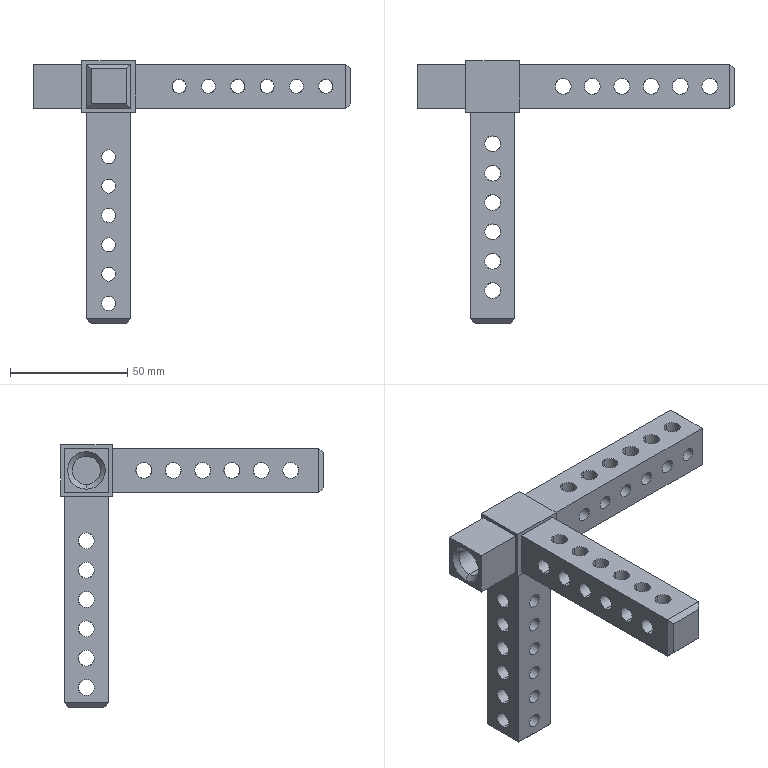Component | SolidWorks | CabinetFrameWeldmentDrawingPG50-01-00-1_FrameConnectionTee1(PG50-01-103-1 | 1 solid | 168 faces | box 135 x 112 x 112 mm | volume 94075 mm3 | cylinder 122 | plane 44 | cone 2 | commonest cylinder face diameters 6.8 x72 6 x48 12 x2 | material AISI 1045 Steel, cold drawn
build123d program:
from build123d import *

# Parameters (mm, degrees)
BOSS_EXTRUDE1_DEPTH      = 9.5
SKETCH2_W                = 19
SKETCH2_H                = 19
BOSS_EXTRUDE2_DEPTH      = 91.5
SKETCH3_W                = 19
SKETCH3_H                = 19
BOSS_EXTRUDE3_DEPTH      = 22.5
SKETCH4_R                = 6
CUT_EXTRUDE1_2_DEPTH     = 20
CHAMFER1_SIZE            = 2
BOSS_EXTRUDE4_DEPTH      = 1.5
BOSS_EXTRUDE4_DEPTH_BACK = 20.5
SKETCH5_W                = 22
SKETCH5_H                = 23
CHAMFER3_SIZE            = 2
SKETCH7_R                = 3.4
CUT_EXTRUDE2_DEPTH       = 183.315
SKETCH8_R                = 3.4
CUT_EXTRUDE3_DEPTH       = 188.263
SKETCH9_R                = 3
CUT_EXTRUDE4_DEPTH       = 188.263
SKETCH1_W                = 23
SKETCH1_H                = 23
SKETCH1_W_2              = 19.2
SKETCH1_H_2              = 19.2
CUT_EXTRUDE1_DEPTH       = 0.02


with BuildPart() as part:
    # Sketch1_2 → Boss-Extrude1 (new, symmetric)
    with BuildSketch(Plane.XY):
        Polygon((0, 0), (110.5, 0), (110.5, -19), (19, -19), (19, -112.5), (0, -112.5), align=None)
    extrude(amount=BOSS_EXTRUDE1_DEPTH, both=True)

    # Sketch2 → Boss-Extrude2 (add)
    with BuildSketch(Plane.XY.offset(9.5)):
        with Locations((9.5, -9.5)):
            Rectangle(SKETCH2_W, SKETCH2_H)
    extrude(amount=BOSS_EXTRUDE2_DEPTH)

    # Sketch3 → Boss-Extrude3 (add)
    with BuildSketch(Plane(origin=(0, 0, 0), x_dir=(1, 0, 0), z_dir=(0, 1, 0))):
        with Locations((9.5, 0)):
            Rectangle(SKETCH3_W, SKETCH3_H)
    extrude(amount=BOSS_EXTRUDE3_DEPTH)

    # Sketch4 → Cut-Extrude1_2 (cut)
    with BuildSketch(Plane(origin=(0, 22.5, 0), x_dir=(1, 0, 0), z_dir=(0, 1, 0))):
        with Locations(Location((9.5, 0, 0), (0, 0, 270))):
            Circle(SKETCH4_R)
    extrude(amount=-CUT_EXTRUDE1_2_DEPTH, mode=Mode.SUBTRACT)

    # Chamfer1
    chamfer1_edges = [part.edges().sort_by_distance(p)[0] for p in [
        (9.5, 22.5, -6),
    ]]
    chamfer(chamfer1_edges, length=CHAMFER1_SIZE)

    # Sketch5 → Boss-Extrude4 (add, two sides: drawn at the far end of the back side and taken through both)
    with BuildSketch(Plane.XY.offset(9.5).offset(-BOSS_EXTRUDE4_DEPTH_BACK)):
        with Locations((9.5, -9.5)):
            Rectangle(SKETCH5_W, SKETCH5_H)
    extrude(amount=BOSS_EXTRUDE4_DEPTH + BOSS_EXTRUDE4_DEPTH_BACK)

    # Chamfer3
    chamfer3_edges = [part.edges().sort_by_distance(p)[0] for p in [
        (110.5, 0, 0),
        (110.5, -19, 0),
        (19, -112.5, 0),
        (0, -112.5, 0),
        (110.5, -9.5, 9.5),
        (0, -9.5, 101),
        (9.5, -19, 101),
        (19, -9.5, 101),
        (9.5, 0, 101),
        (110.5, -9.5, -9.5),
        (9.5, -112.5, 9.5),
        (9.5, -112.5, -9.5),
    ]]
    chamfer(chamfer3_edges, length=CHAMFER3_SIZE)

    # Sketch7 → Cut-Extrude2 (cut, through all)
    with BuildSketch(Plane.XY.offset(9.5)):
        with Locations((96.5, -9.5)):
            Circle(SKETCH7_R)
        with Locations((84, -9.5)):
            Circle(SKETCH7_R)
        with Locations((71.5, -9.5)):
            Circle(SKETCH7_R)
        with Locations((59, -9.5)):
            Circle(SKETCH7_R)
        with Locations((46.5, -9.5)):
            Circle(SKETCH7_R)
        with Locations((34, -9.5)):
            Circle(SKETCH7_R)
        with Locations((9.5, -102)):
            Circle(SKETCH7_R)
        with Locations((9.5, -89.5)):
            Circle(SKETCH7_R)
        with Locations((9.5, -77)):
            Circle(SKETCH7_R)
        with Locations((9.5, -64.5)):
            Circle(SKETCH7_R)
        with Locations((9.5, -52)):
            Circle(SKETCH7_R)
        with Locations((9.5, -39.5)):
            Circle(SKETCH7_R)
    extrude(amount=-CUT_EXTRUDE2_DEPTH, mode=Mode.SUBTRACT)

    # Sketch8 → Cut-Extrude3 (cut, through all)
    with BuildSketch(Plane(origin=(0, 0, 0), x_dir=(1, 0, 0), z_dir=(0, 1, 0))):
        with Locations(Location((9.5, -92.5, 0), (0, 0, 270))):
            Circle(SKETCH8_R)
        with Locations(Location((9.5, -80, 0), (0, 0, 270))):
            Circle(SKETCH8_R)
        with Locations(Location((9.5, -67.5, 0), (0, 0, 270))):
            Circle(SKETCH8_R)
        with Locations(Location((9.5, -55, 0), (0, 0, 270))):
            Circle(SKETCH8_R)
        with Locations(Location((9.5, -42.5, 0), (0, 0, 270))):
            Circle(SKETCH8_R)
        with Locations(Location((96.5, 0, 0), (0, 0, 270))):
            Circle(SKETCH8_R)
        with Locations(Location((84, 0, 0), (0, 0, 270))):
            Circle(SKETCH8_R)
        with Locations(Location((71.5, 0, 0), (0, 0, 270))):
            Circle(SKETCH8_R)
        with Locations(Location((59, 0, 0), (0, 0, 270))):
            Circle(SKETCH8_R)
        with Locations(Location((46.5, 0, 0), (0, 0, 270))):
            Circle(SKETCH8_R)
        with Locations(Location((34, 0, 0), (0, 0, 270))):
            Circle(SKETCH8_R)
        with Locations(Location((9.5, -30, 0), (0, 0, 270))):
            Circle(SKETCH8_R)
    extrude(amount=-CUT_EXTRUDE3_DEPTH, mode=Mode.SUBTRACT)

    # Sketch9 → Cut-Extrude4 (cut, through all)
    with BuildSketch(Plane.ZY):
        with Locations(Location((30, -9.5, 0), (0, 0, 270))):
            Circle(SKETCH9_R)
        with Locations(Location((42.5, -9.5, 0), (0, 0, 270))):
            Circle(SKETCH9_R)
        with Locations(Location((55, -9.5, 0), (0, 0, 270))):
            Circle(SKETCH9_R)
        with Locations(Location((67.5, -9.5, 0), (0, 0, 270))):
            Circle(SKETCH9_R)
        with Locations(Location((80, -9.5, 0), (0, 0, 270))):
            Circle(SKETCH9_R)
        with Locations(Location((92.5, -9.5, 0), (0, 0, 270))):
            Circle(SKETCH9_R)
        with Locations(Location((0, -39.5, 0), (0, 0, 270))):
            Circle(SKETCH9_R)
        with Locations(Location((0, -52, 0), (0, 0, 270))):
            Circle(SKETCH9_R)
        with Locations(Location((0, -64.5, 0), (0, 0, 270))):
            Circle(SKETCH9_R)
        with Locations(Location((0, -77, 0), (0, 0, 270))):
            Circle(SKETCH9_R)
        with Locations(Location((0, -89.5, 0), (0, 0, 270))):
            Circle(SKETCH9_R)
        with Locations(Location((0, -102, 0), (0, 0, 270))):
            Circle(SKETCH9_R)
    extrude(amount=-CUT_EXTRUDE4_DEPTH, mode=Mode.SUBTRACT)

    # Sketch1 → Cut-Extrude1 (cut)
    with BuildSketch(Plane.XZ.offset(21)):
        with Locations((9.5, 0)):
            Rectangle(SKETCH1_W, SKETCH1_H)
        with Locations((9.5, 0)):
            Rectangle(SKETCH1_W_2, SKETCH1_H_2, mode=Mode.SUBTRACT)
    extrude(amount=-CUT_EXTRUDE1_DEPTH, mode=Mode.SUBTRACT)


solid = part.part

# Placed as in the assembly
solid = solid.moved(Location((-1150.67, 286.707, 367.503), (180, 0, 90)))